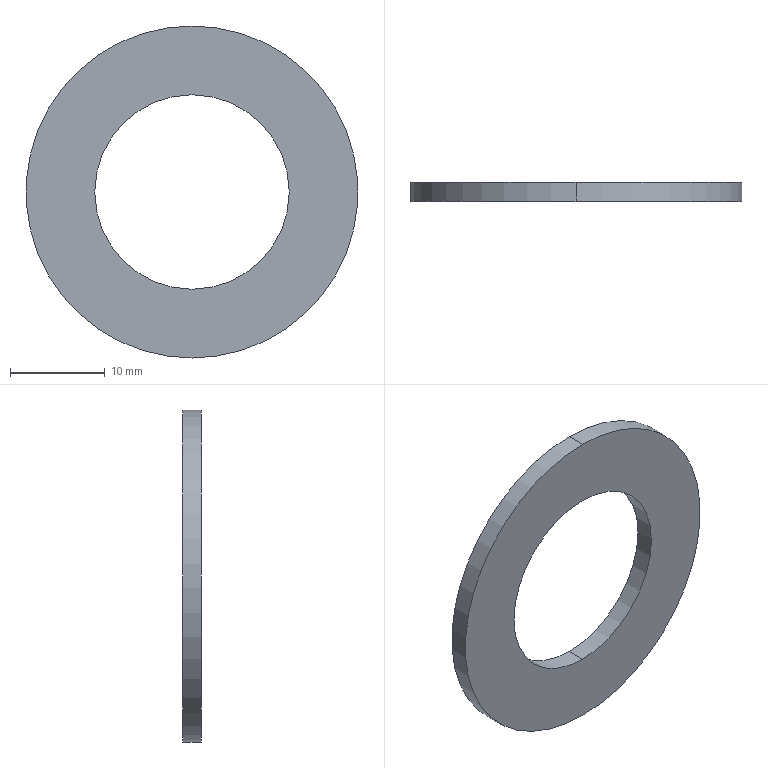Component | SolidWorks | 8TC-A15004-40-25A-1 | 1 solid | 6 faces | box 35 x 2 x 35 mm | volume 1264 mm3 | cylinder 4 | plane 2 | commonest cylinder face diameters 20.5 x2 35 x2 | material A3
build123d program:
from build123d import *

# Parameters (mm, degrees)
SKETCH1_R           = 17.5
SKETCH1_R_2         = 10.25
BOSS_EXTRUDE1_DEPTH = 1


with BuildPart() as part:
    # Sketch1 → Boss-Extrude1 (new, symmetric)
    with BuildSketch(Plane(origin=(0, 0, 0), x_dir=(1, 0, 0), z_dir=(0, 1, 0))):
        with Locations(Location((0, 0, 0), (0, 0, 270))):
            Circle(SKETCH1_R)
        with Locations(Location((0, 0, 0), (0, 0, 270))):
            Circle(SKETCH1_R_2, mode=Mode.SUBTRACT)
    extrude(amount=BOSS_EXTRUDE1_DEPTH, both=True)


solid = part.part

# Placed as in the assembly
solid = solid.moved(Location((40, 21.5, -750), (0, 0, 0)))
STEP:
#1=COLOUR_RGB('',0.7922,0.8196,0.9333);
#2=FILL_AREA_STYLE_COLOUR('',#1);
#3=FILL_AREA_STYLE('',(#2));
#4=SURFACE_STYLE_FILL_AREA(#3);
#5=SURFACE_SIDE_STYLE('',(#4));
#6=SURFACE_STYLE_USAGE(.BOTH.,#5);
#7=PRESENTATION_STYLE_ASSIGNMENT((#6));
#8=CARTESIAN_POINT('',(1.575,0.8858,-29.931));
#9=VERTEX_POINT('',#8);
#10=CARTESIAN_POINT('',(1.575,0.8858,-29.124));
#11=VERTEX_POINT('',#10);
#12=CARTESIAN_POINT('',(1.575,0.8858,-29.528));
#13=DIRECTION('',(0.,1.,0.));
#14=DIRECTION('',(0.,0.,1.));
#15=AXIS2_PLACEMENT_3D('',#12,#13,#14);
#16=CIRCLE('',#15,0.4035);
#17=EDGE_CURVE('',#9,#11,#16,.T.);
#18=ORIENTED_EDGE('',*,*,#17,.T.);
#19=CARTESIAN_POINT('',(1.575,0.8071,-29.124));
#20=VERTEX_POINT('',#19);
#21=CARTESIAN_POINT('',(1.575,0.8858,-29.124));
#22=DIRECTION('',(0.,-1.,0.));
#23=VECTOR('',#22,39.37);
#24=LINE('',#21,#23);
#25=EDGE_CURVE('',#11,#20,#24,.T.);
#26=ORIENTED_EDGE('',*,*,#25,.T.);
#27=CARTESIAN_POINT('',(1.575,0.8071,-29.931));
#28=VERTEX_POINT('',#27);
#29=CARTESIAN_POINT('',(1.575,0.8071,-29.528));
#30=DIRECTION('',(0.,1.,0.));
#31=DIRECTION('',(0.,0.,1.));
#32=AXIS2_PLACEMENT_3D('',#29,#30,#31);
#33=CIRCLE('',#32,0.4035);
#34=EDGE_CURVE('',#28,#20,#33,.T.);
#35=ORIENTED_EDGE('',*,*,#34,.F.);
#36=CARTESIAN_POINT('',(1.575,0.8858,-29.931));
#37=DIRECTION('',(0.,-1.,0.));
#38=VECTOR('',#37,39.37);
#39=LINE('',#36,#38);
#40=EDGE_CURVE('',#9,#28,#39,.T.);
#41=ORIENTED_EDGE('',*,*,#40,.F.);
#42=EDGE_LOOP('',(#18,#26,#35,#41));
#43=FACE_OUTER_BOUND('',#42,.T.);
#44=CARTESIAN_POINT('',(1.575,0.8858,-29.528));
#45=DIRECTION('',(0.,-1.,0.));
#46=DIRECTION('',(0.,0.,-1.));
#47=AXIS2_PLACEMENT_3D('',#44,#45,#46);
#48=CYLINDRICAL_SURFACE('',#47,0.4035);
#49=ADVANCED_FACE('',(#43),#48,.F.);
#50=CARTESIAN_POINT('',(1.575,0.8858,-28.839));
#51=VERTEX_POINT('',#50);
#52=CARTESIAN_POINT('',(1.575,0.8858,-30.217));
#53=VERTEX_POINT('',#52);
#54=CARTESIAN_POINT('',(1.575,0.8858,-29.528));
#55=DIRECTION('',(0.,1.,0.));
#56=DIRECTION('',(0.,0.,1.));
#57=AXIS2_PLACEMENT_3D('',#54,#55,#56);
#58=CIRCLE('',#57,0.689);
#59=EDGE_CURVE('',#51,#53,#58,.T.);
#60=ORIENTED_EDGE('',*,*,#59,.F.);
#61=CARTESIAN_POINT('',(1.575,0.8071,-28.839));
#62=VERTEX_POINT('',#61);
#63=CARTESIAN_POINT('',(1.575,0.8858,-28.839));
#64=DIRECTION('',(0.,-1.,0.));
#65=VECTOR('',#64,39.37);
#66=LINE('',#63,#65);
#67=EDGE_CURVE('',#51,#62,#66,.T.);
#68=ORIENTED_EDGE('',*,*,#67,.T.);
#69=CARTESIAN_POINT('',(1.575,0.8071,-30.217));
#70=VERTEX_POINT('',#69);
#71=CARTESIAN_POINT('',(1.575,0.8071,-29.528));
#72=DIRECTION('',(0.,1.,0.));
#73=DIRECTION('',(0.,0.,1.));
#74=AXIS2_PLACEMENT_3D('',#71,#72,#73);
#75=CIRCLE('',#74,0.689);
#76=EDGE_CURVE('',#62,#70,#75,.T.);
#77=ORIENTED_EDGE('',*,*,#76,.T.);
#78=CARTESIAN_POINT('',(1.575,0.8858,-30.217));
#79=DIRECTION('',(0.,-1.,0.));
#80=VECTOR('',#79,39.37);
#81=LINE('',#78,#80);
#82=EDGE_CURVE('',#53,#70,#81,.T.);
#83=ORIENTED_EDGE('',*,*,#82,.F.);
#84=EDGE_LOOP('',(#60,#68,#77,#83));
#85=FACE_OUTER_BOUND('',#84,.T.);
#86=CARTESIAN_POINT('',(1.575,0.8858,-29.528));
#87=DIRECTION('',(0.,-1.,0.));
#88=DIRECTION('',(0.,0.,-1.));
#89=AXIS2_PLACEMENT_3D('',#86,#87,#88);
#90=CYLINDRICAL_SURFACE('',#89,0.689);
#91=ADVANCED_FACE('',(#85),#90,.T.);
#92=CARTESIAN_POINT('',(1.575,0.8858,-29.528));
#93=DIRECTION('',(0.,1.,0.));
#94=DIRECTION('',(0.,0.,1.));
#95=AXIS2_PLACEMENT_3D('',#92,#93,#94);
#96=CIRCLE('',#95,0.689);
#97=EDGE_CURVE('',#53,#51,#96,.T.);
#98=ORIENTED_EDGE('',*,*,#97,.T.);
#99=ORIENTED_EDGE('',*,*,#59,.T.);
#100=EDGE_LOOP('',(#98,#99));
#101=FACE_OUTER_BOUND('',#100,.T.);
#102=ORIENTED_EDGE('',*,*,#17,.F.);
#103=CARTESIAN_POINT('',(1.575,0.8858,-29.528));
#104=DIRECTION('',(0.,1.,0.));
#105=DIRECTION('',(0.,0.,1.));
#106=AXIS2_PLACEMENT_3D('',#103,#104,#105);
#107=CIRCLE('',#106,0.4035);
#108=EDGE_CURVE('',#11,#9,#107,.T.);
#109=ORIENTED_EDGE('',*,*,#108,.F.);
#110=EDGE_LOOP('',(#102,#109));
#111=FACE_BOUND('',#110,.T.);
#112=CARTESIAN_POINT('',(1.575,0.8858,-29.528));
#113=DIRECTION('',(0.,1.,0.));
#114=DIRECTION('',(0.,0.,1.));
#115=AXIS2_PLACEMENT_3D('',#112,#113,#114);
#116=PLANE('',#115);
#117=ADVANCED_FACE('',(#101,#111),#116,.T.);
#118=CARTESIAN_POINT('',(1.575,0.8071,-29.528));
#119=DIRECTION('',(0.,1.,0.));
#120=DIRECTION('',(0.,0.,1.));
#121=AXIS2_PLACEMENT_3D('',#118,#119,#120);
#122=CIRCLE('',#121,0.689);
#123=EDGE_CURVE('',#70,#62,#122,.T.);
#124=ORIENTED_EDGE('',*,*,#123,.F.);
#125=ORIENTED_EDGE('',*,*,#76,.F.);
#126=EDGE_LOOP('',(#124,#125));
#127=FACE_OUTER_BOUND('',#126,.T.);
#128=ORIENTED_EDGE('',*,*,#34,.T.);
#129=CARTESIAN_POINT('',(1.575,0.8071,-29.528));
#130=DIRECTION('',(0.,1.,0.));
#131=DIRECTION('',(0.,0.,1.));
#132=AXIS2_PLACEMENT_3D('',#129,#130,#131);
#133=CIRCLE('',#132,0.4035);
#134=EDGE_CURVE('',#20,#28,#133,.T.);
#135=ORIENTED_EDGE('',*,*,#134,.T.);
#136=EDGE_LOOP('',(#128,#135));
#137=FACE_BOUND('',#136,.T.);
#138=CARTESIAN_POINT('',(1.575,0.8071,-29.528));
#139=DIRECTION('',(0.,1.,0.));
#140=DIRECTION('',(0.,0.,1.));
#141=AXIS2_PLACEMENT_3D('',#138,#139,#140);
#142=PLANE('',#141);
#143=ADVANCED_FACE('',(#127,#137),#142,.F.);
#144=ORIENTED_EDGE('',*,*,#67,.F.);
#145=ORIENTED_EDGE('',*,*,#97,.F.);
#146=ORIENTED_EDGE('',*,*,#82,.T.);
#147=ORIENTED_EDGE('',*,*,#123,.T.);
#148=EDGE_LOOP('',(#144,#145,#146,#147));
#149=FACE_OUTER_BOUND('',#148,.T.);
#150=CARTESIAN_POINT('',(1.575,0.8858,-29.528));
#151=DIRECTION('',(0.,-1.,0.));
#152=DIRECTION('',(0.,0.,-1.));
#153=AXIS2_PLACEMENT_3D('',#150,#151,#152);
#154=CYLINDRICAL_SURFACE('',#153,0.689);
#155=ADVANCED_FACE('',(#149),#154,.T.);
#156=ORIENTED_EDGE('',*,*,#25,.F.);
#157=ORIENTED_EDGE('',*,*,#108,.T.);
#158=ORIENTED_EDGE('',*,*,#40,.T.);
#159=ORIENTED_EDGE('',*,*,#134,.F.);
#160=EDGE_LOOP('',(#156,#157,#158,#159));
#161=FACE_OUTER_BOUND('',#160,.T.);
#162=CARTESIAN_POINT('',(1.575,0.8858,-29.528));
#163=DIRECTION('',(0.,-1.,0.));
#164=DIRECTION('',(0.,0.,-1.));
#165=AXIS2_PLACEMENT_3D('',#162,#163,#164);
#166=CYLINDRICAL_SURFACE('',#165,0.4035);
#167=ADVANCED_FACE('',(#161),#166,.F.);
#168=CLOSED_SHELL('',(#49,#91,#117,#143,#155,#167));
#169=MANIFOLD_SOLID_BREP('',#168);
#170=STYLED_ITEM('',(#7),#169);
#171=PRESENTATION_LAYER_ASSIGNMENT('','',(#170));
#172=CARTESIAN_POINT('',(0.,0.,0.));
#173=DIRECTION('',(0.,0.,1.));
#174=DIRECTION('',(1.,0.,0.));
#175=AXIS2_PLACEMENT_3D('',#172,#173,#174);
#176=(LENGTH_UNIT()NAMED_UNIT(*)SI_UNIT($,.METRE.));
#177=LENGTH_MEASURE_WITH_UNIT(LENGTH_MEASURE(0.0254),#176);
#178=DIMENSIONAL_EXPONENTS(1.,0.,0.,0.,0.,0.,0.);
#179=(CONVERSION_BASED_UNIT('',#177)LENGTH_UNIT()NAMED_UNIT(#178));
#180=UNCERTAINTY_MEASURE_WITH_UNIT(LENGTH_MEASURE(0.00001),#179,'','');
#181=(NAMED_UNIT(*)PLANE_ANGLE_UNIT()SI_UNIT($,.RADIAN.));
#182=(NAMED_UNIT(*)SI_UNIT($,.STERADIAN.)SOLID_ANGLE_UNIT());
#183=(GEOMETRIC_REPRESENTATION_CONTEXT(3)GLOBAL_UNCERTAINTY_ASSIGNED_CONTEXT((#180))GLOBAL_UNIT_ASSIGNED_CONTEXT((#179,#181,#182))REPRESENTATION_CONTEXT('',''));
#184=ADVANCED_BREP_SHAPE_REPRESENTATION('',(#169,#175),#183);
#185=(LENGTH_UNIT()NAMED_UNIT(*)SI_UNIT($,.METRE.));
#186=LENGTH_MEASURE_WITH_UNIT(LENGTH_MEASURE(0.0254),#185);
#187=DIMENSIONAL_EXPONENTS(1.,0.,0.,0.,0.,0.,0.);
#188=(CONVERSION_BASED_UNIT('',#186)LENGTH_UNIT()NAMED_UNIT(#187));
#189=UNCERTAINTY_MEASURE_WITH_UNIT(LENGTH_MEASURE(0.00001),#188,'','');
#190=(NAMED_UNIT(*)PLANE_ANGLE_UNIT()SI_UNIT($,.RADIAN.));
#191=(NAMED_UNIT(*)SI_UNIT($,.STERADIAN.)SOLID_ANGLE_UNIT());
#192=(GEOMETRIC_REPRESENTATION_CONTEXT(3)GLOBAL_UNCERTAINTY_ASSIGNED_CONTEXT((#189))GLOBAL_UNIT_ASSIGNED_CONTEXT((#188,#190,#191))REPRESENTATION_CONTEXT('',''));
#193=MECHANICAL_DESIGN_GEOMETRIC_PRESENTATION_REPRESENTATION('',(#170),#192);